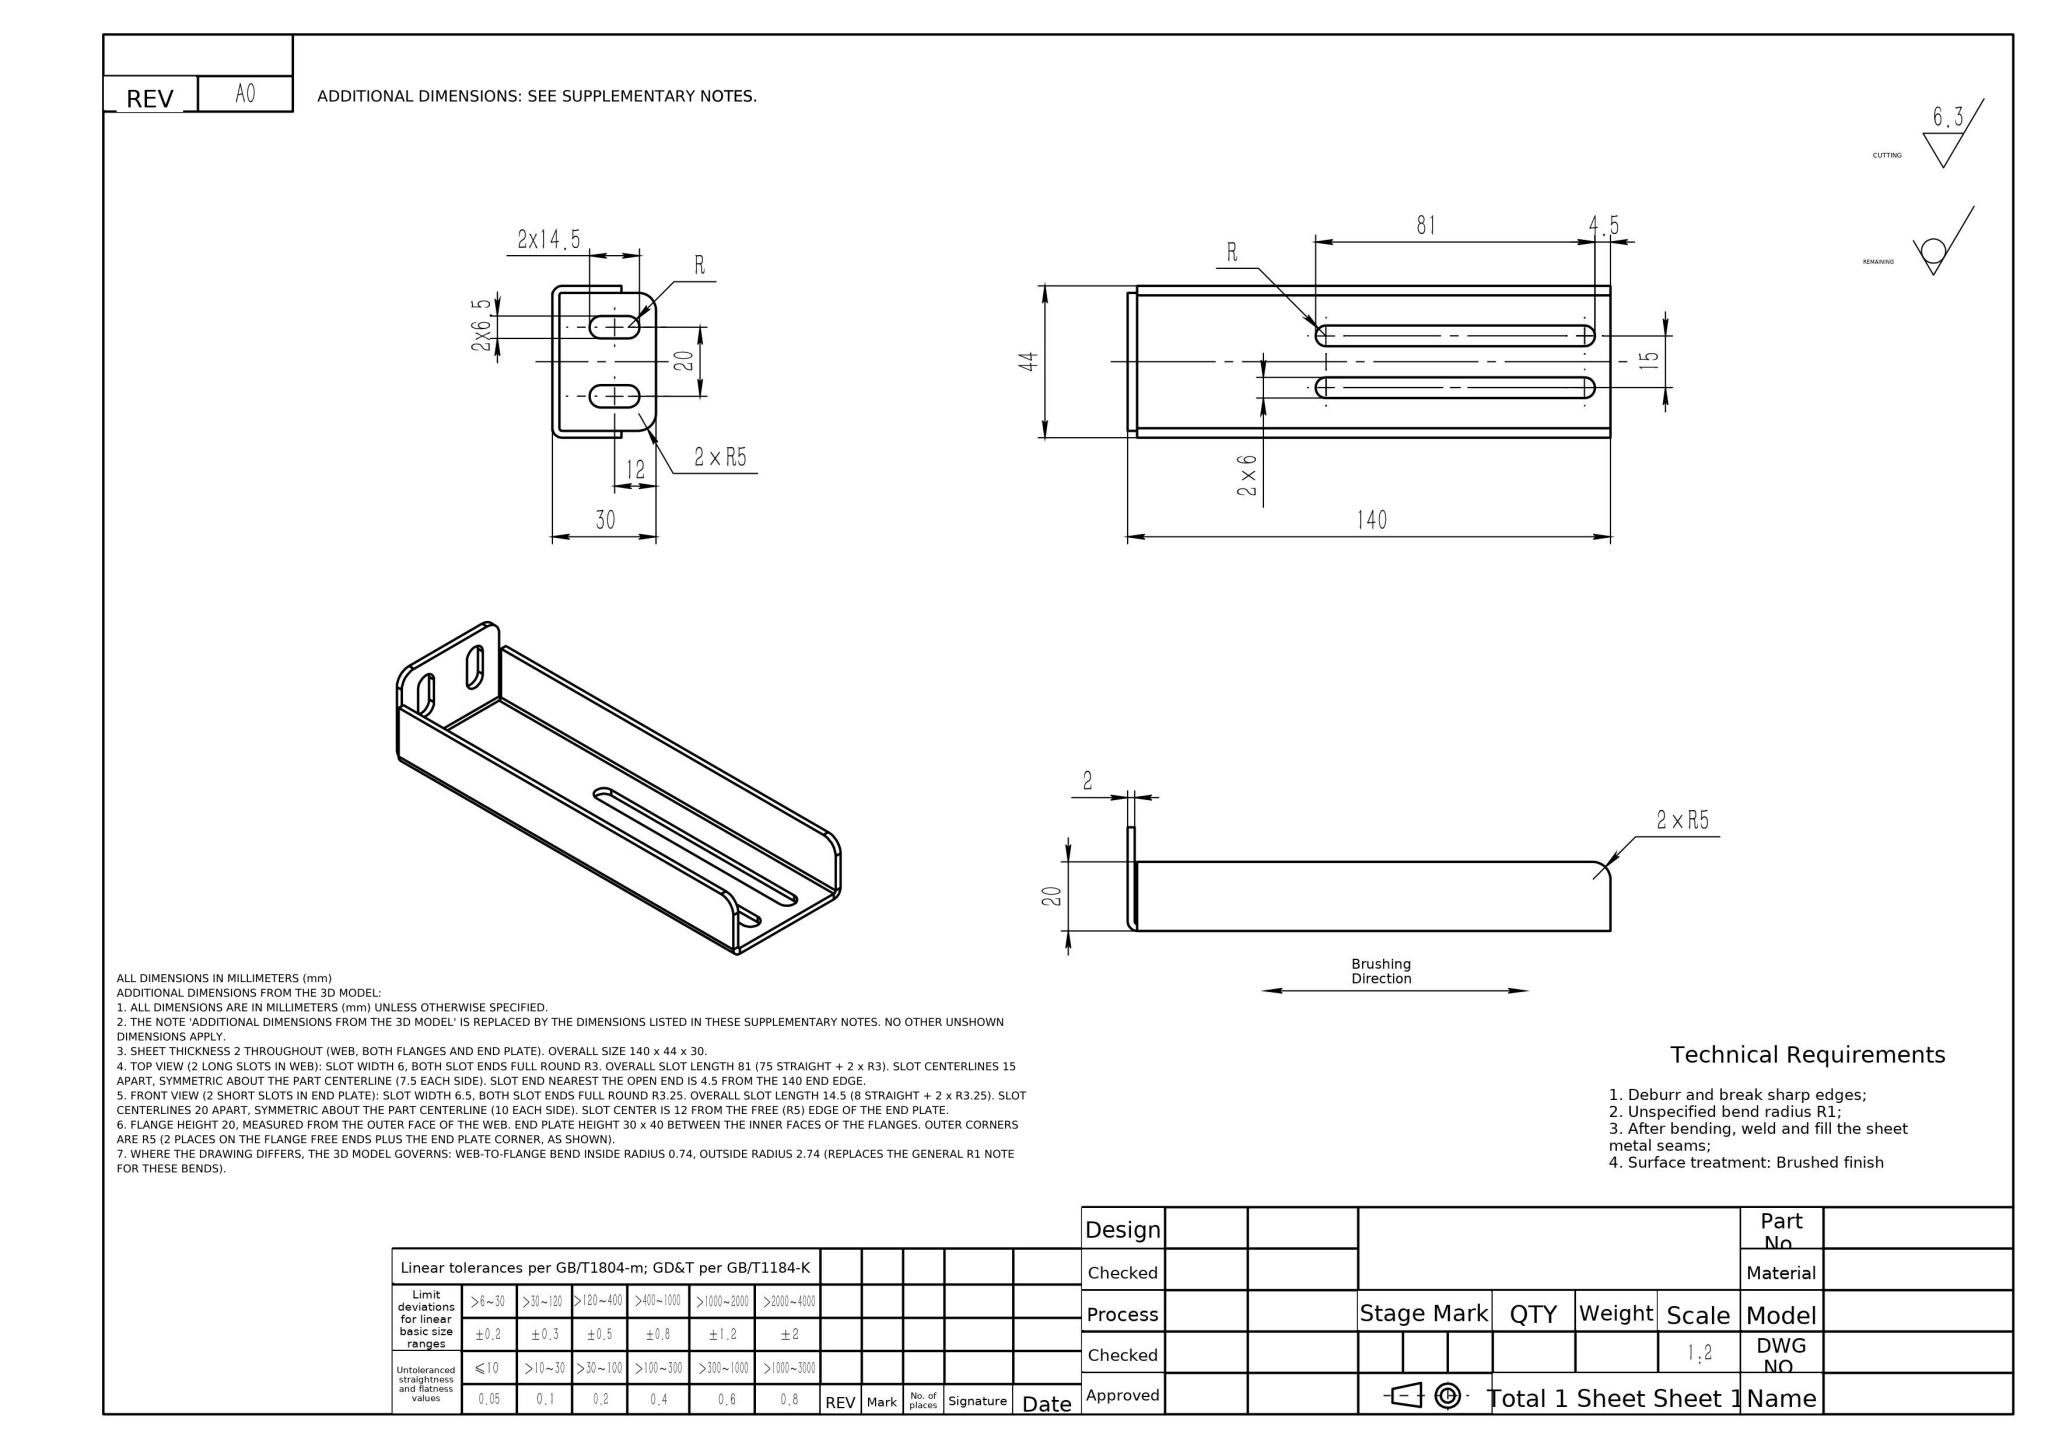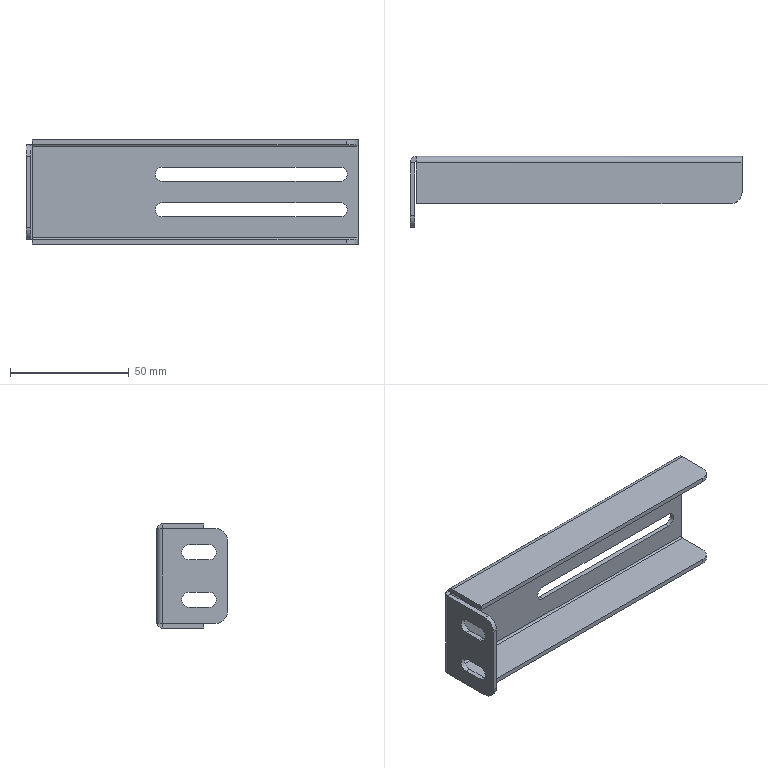Part | NX | mm | Slotted U-Channel Mounting Bracket | 1 solid | 52 faces | box 140 x 30 x 44 mm | volume 21655 mm3 | plane 34 | cylinder 18 | commonest cylinder face diameters 6.5 x4 10 x4 6 x4 5.473 x3 1.473 x3